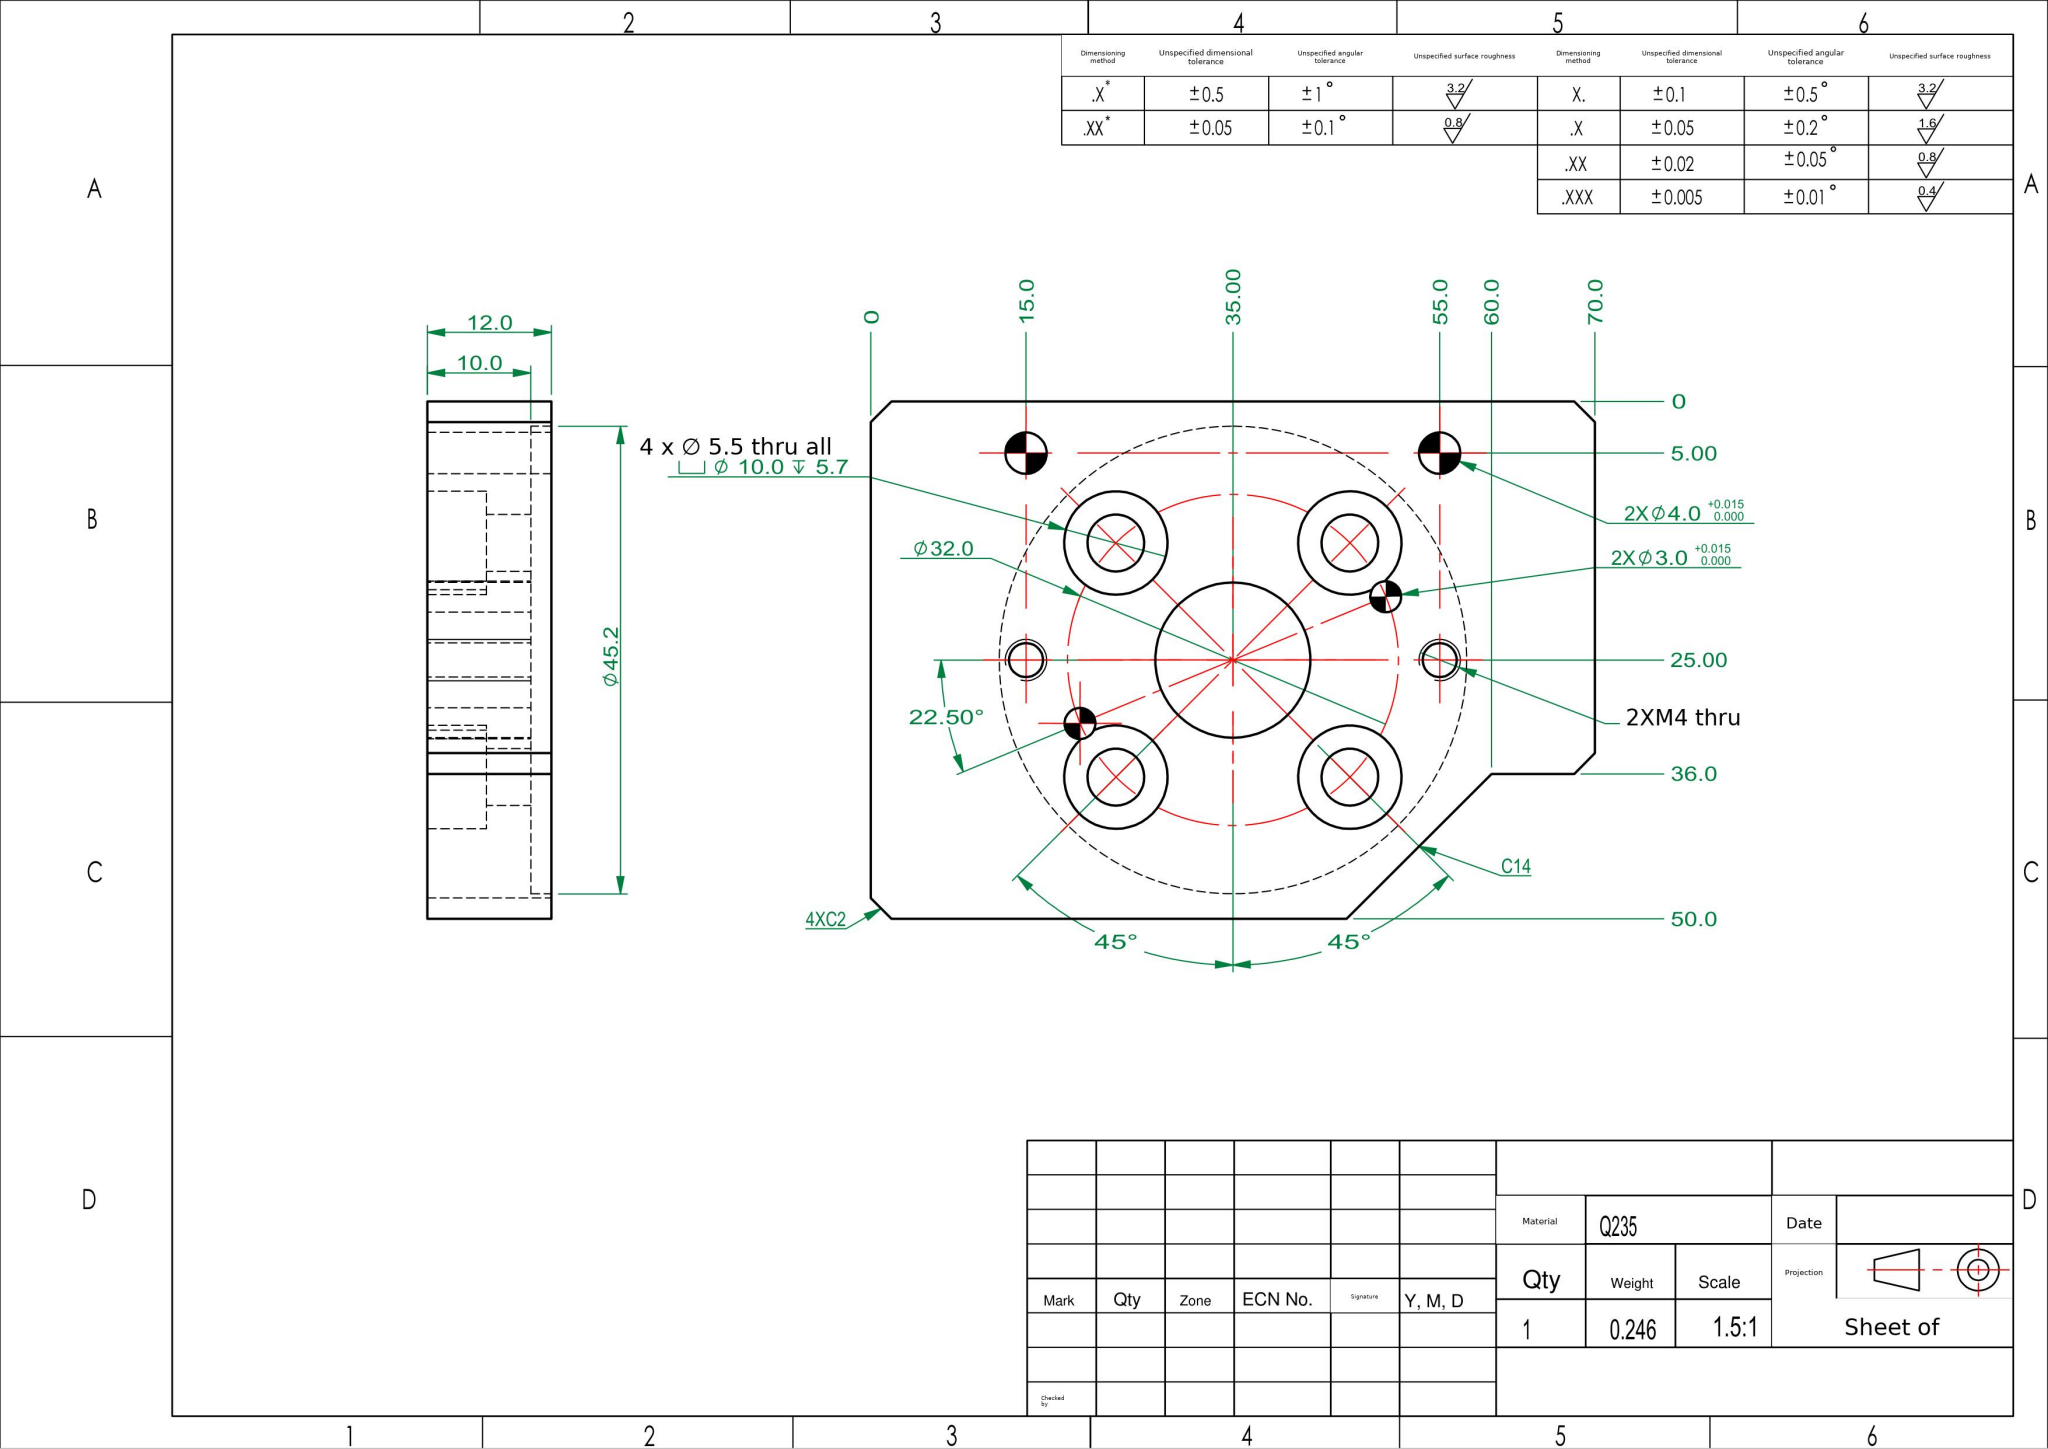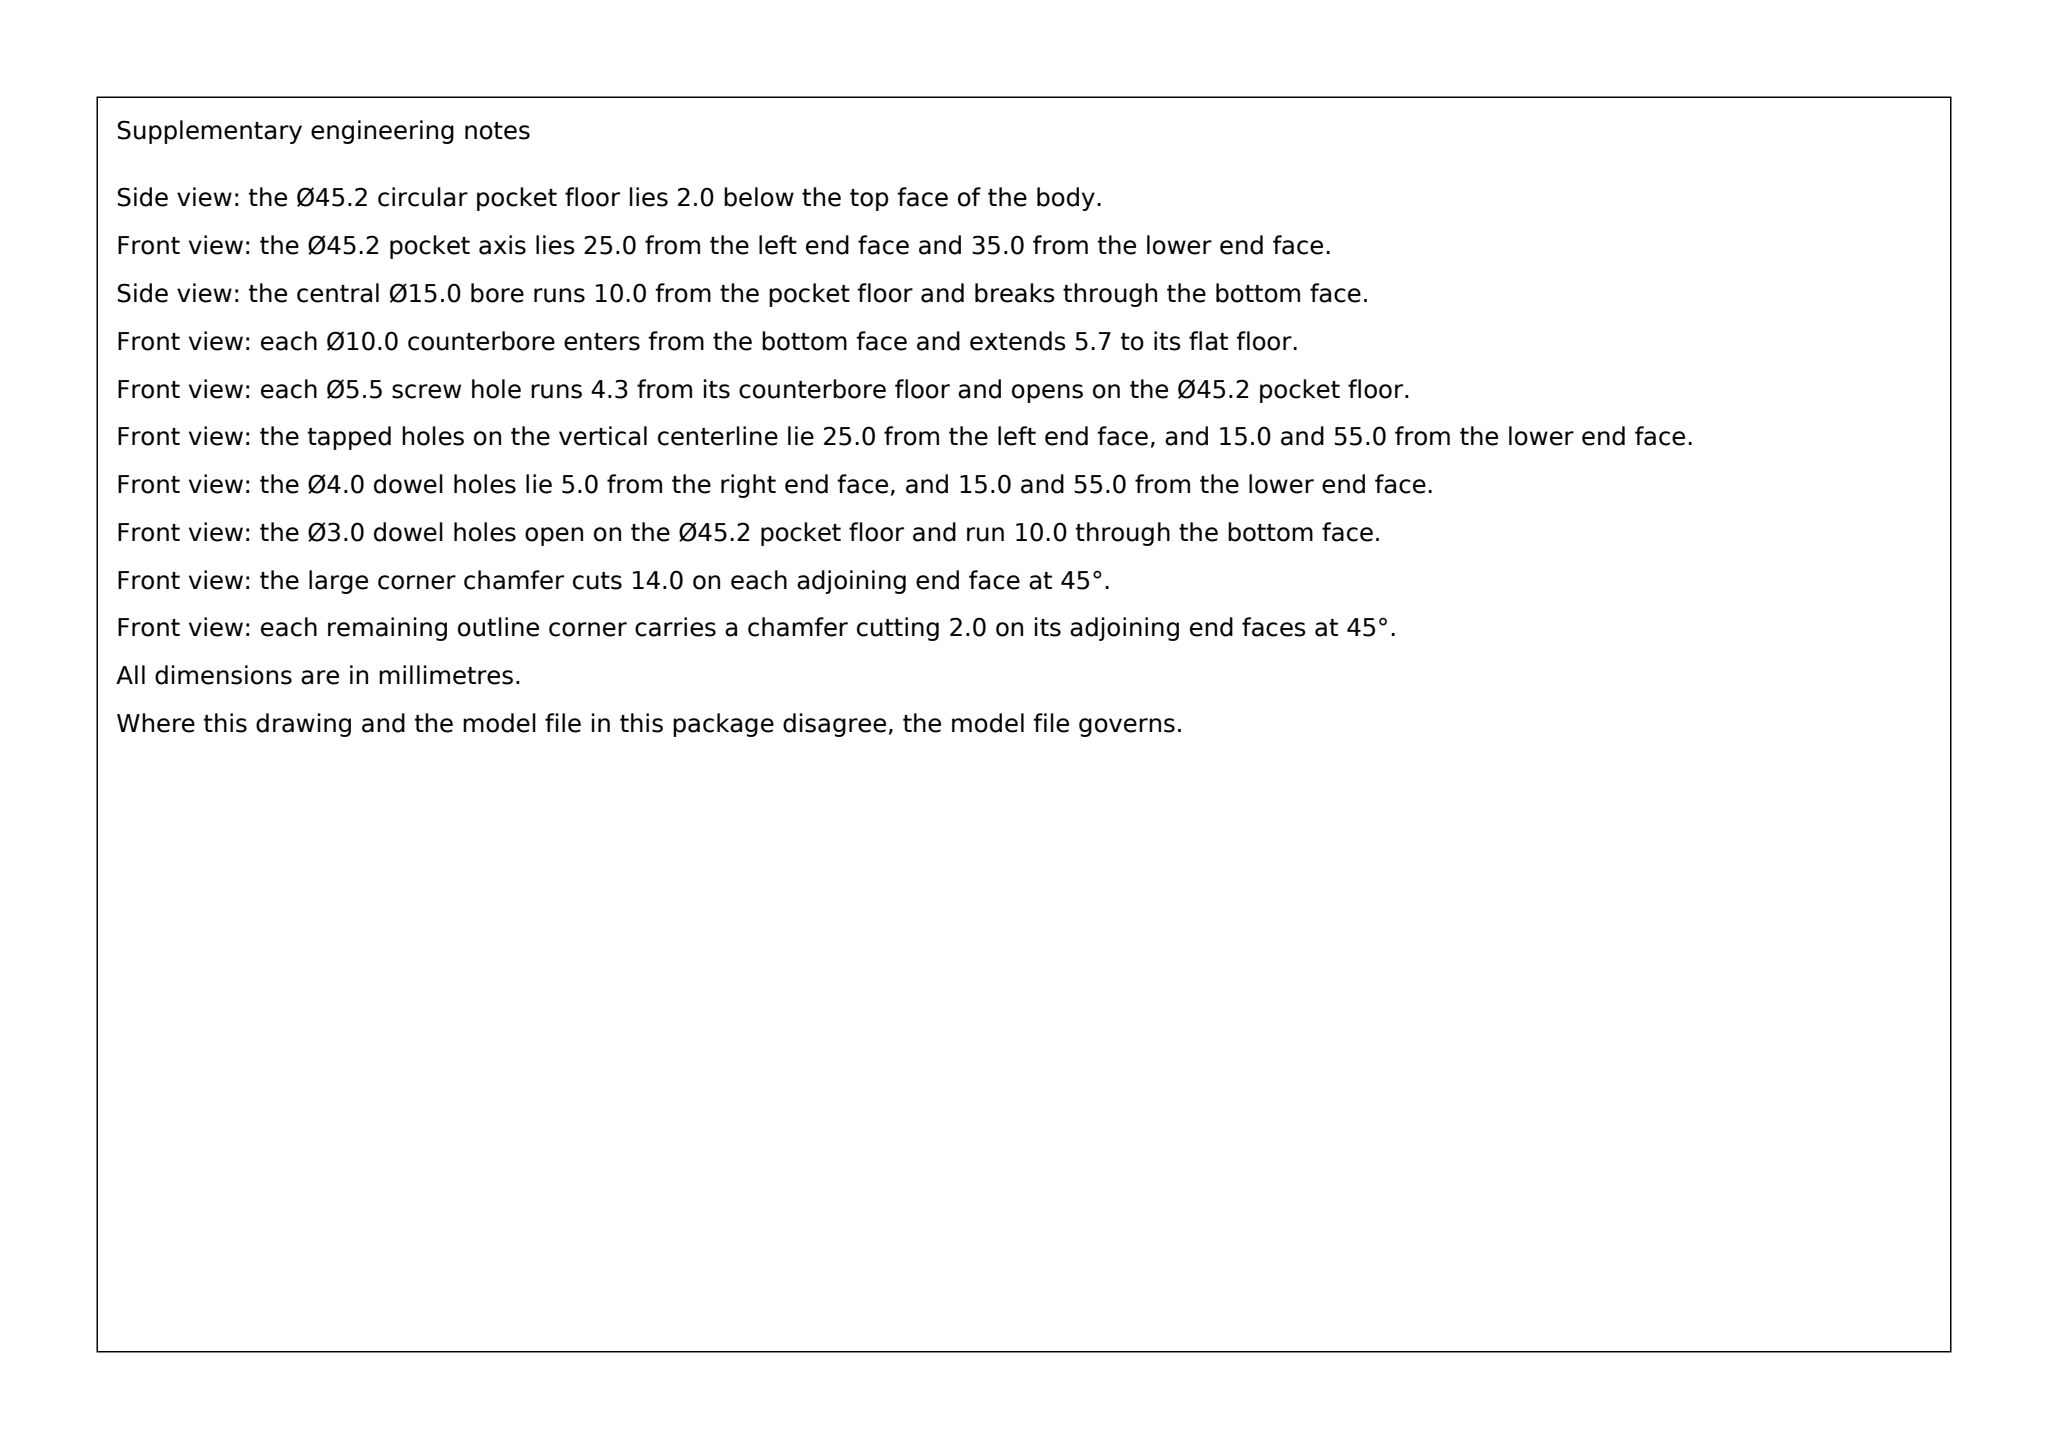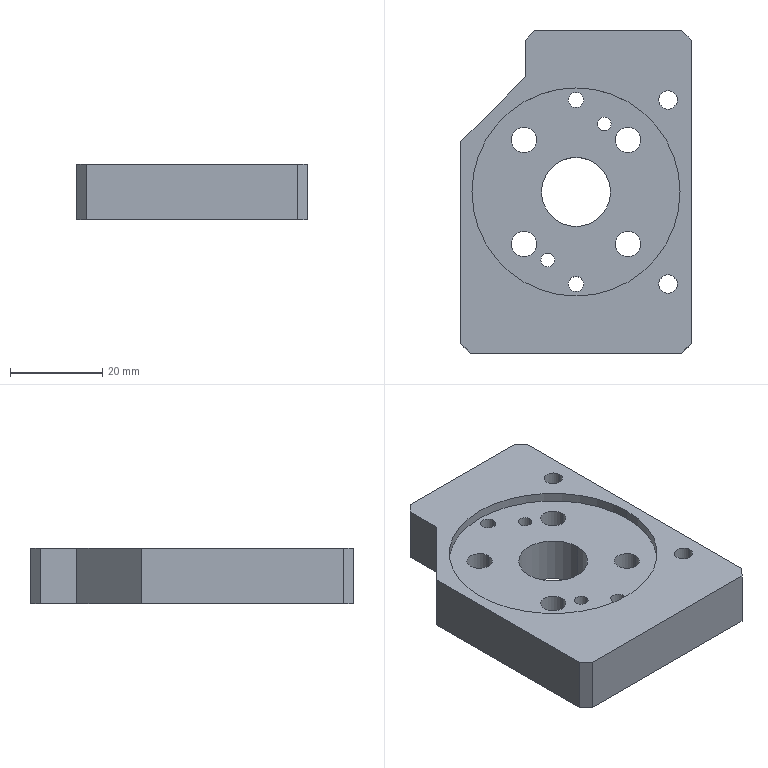Part | SolidWorks | mm | material Q235 | 1 solid | 51 faces | box 50 x 70 x 12 mm | volume 31261 mm3 | cylinder 34 | plane 17 | commonest cylinder face diameters 10 x10 5.5 x8 3 x4 4 x4 3.3 x4 15 x2 45.2 x2
Drawing notes:
Ø15.0 DP 10.0 FROM Ø45.2 POCKET FLOOR, NOT THRU | from the solid: cyl dia 15.0, axis z at (25.0,35.0), length 10.0; Ø45.2 c'bore depth 2.0 of 12.0 thk plate
2X Ø3.0 +0.015/0 DP 10.0 FROM Ø45.2 POCKET FLOOR, NOT THRU | from the solid: 2 cyl dia 3.0, axis z at (18.88,20.22) & (31.12,49.78), length 10.0; plate 12.0 thk
2X Ø4.0 +0.015/0 THRU ALL (12.0) | from the solid: cylinders 4.0 dia, z axis, at (45.0,15.0) and (45.0,55.0), length 12.0 = full bbox thickness 12.0